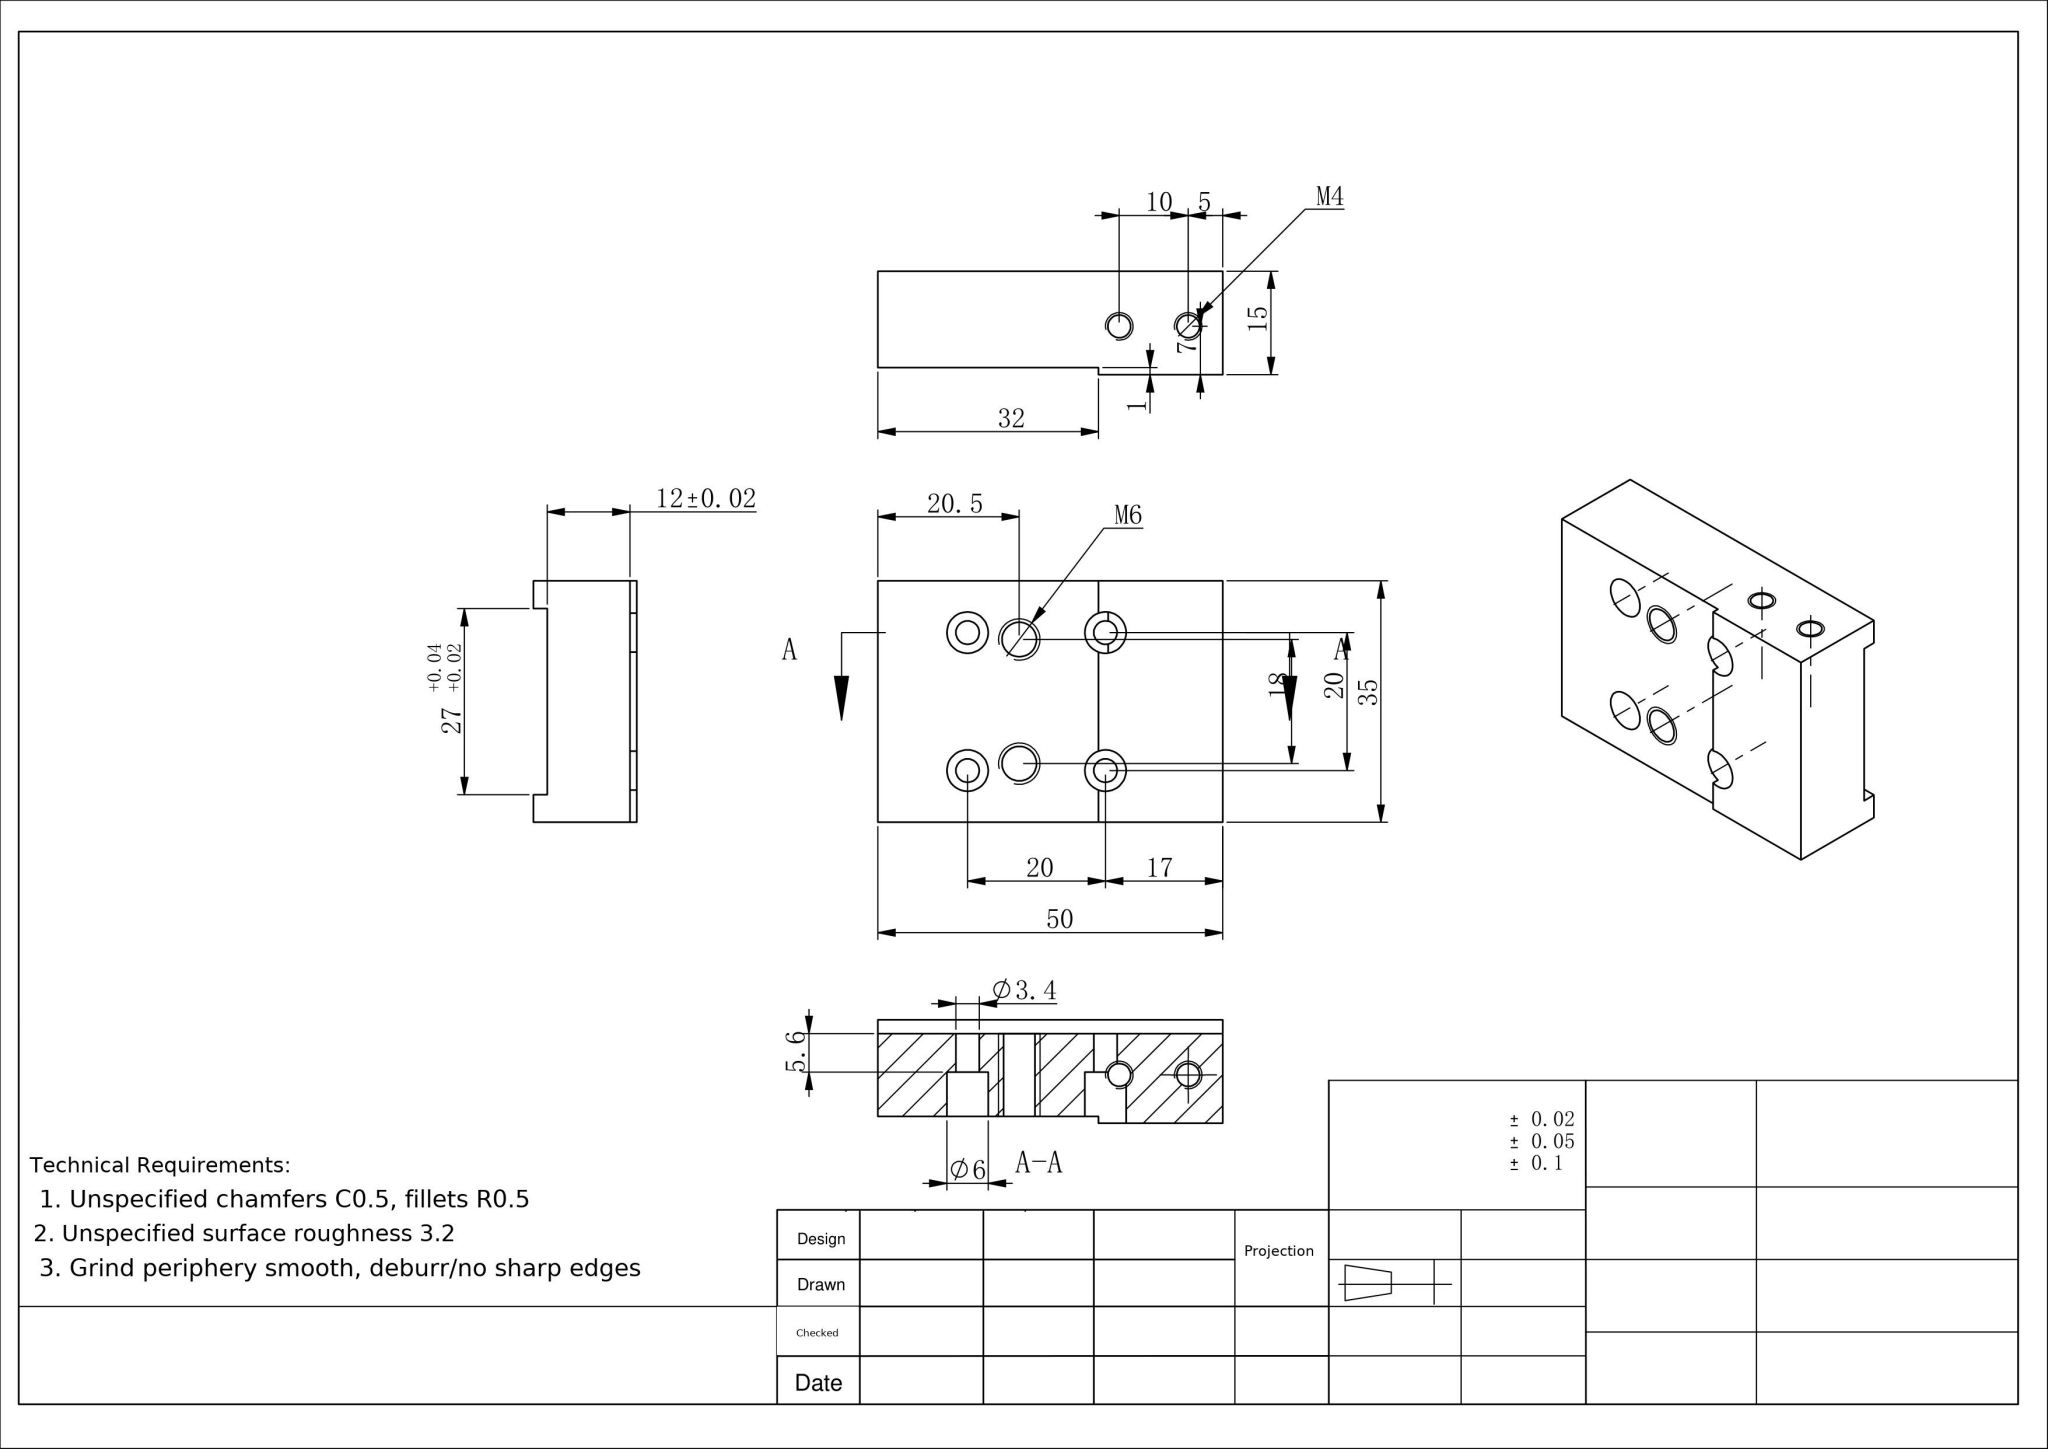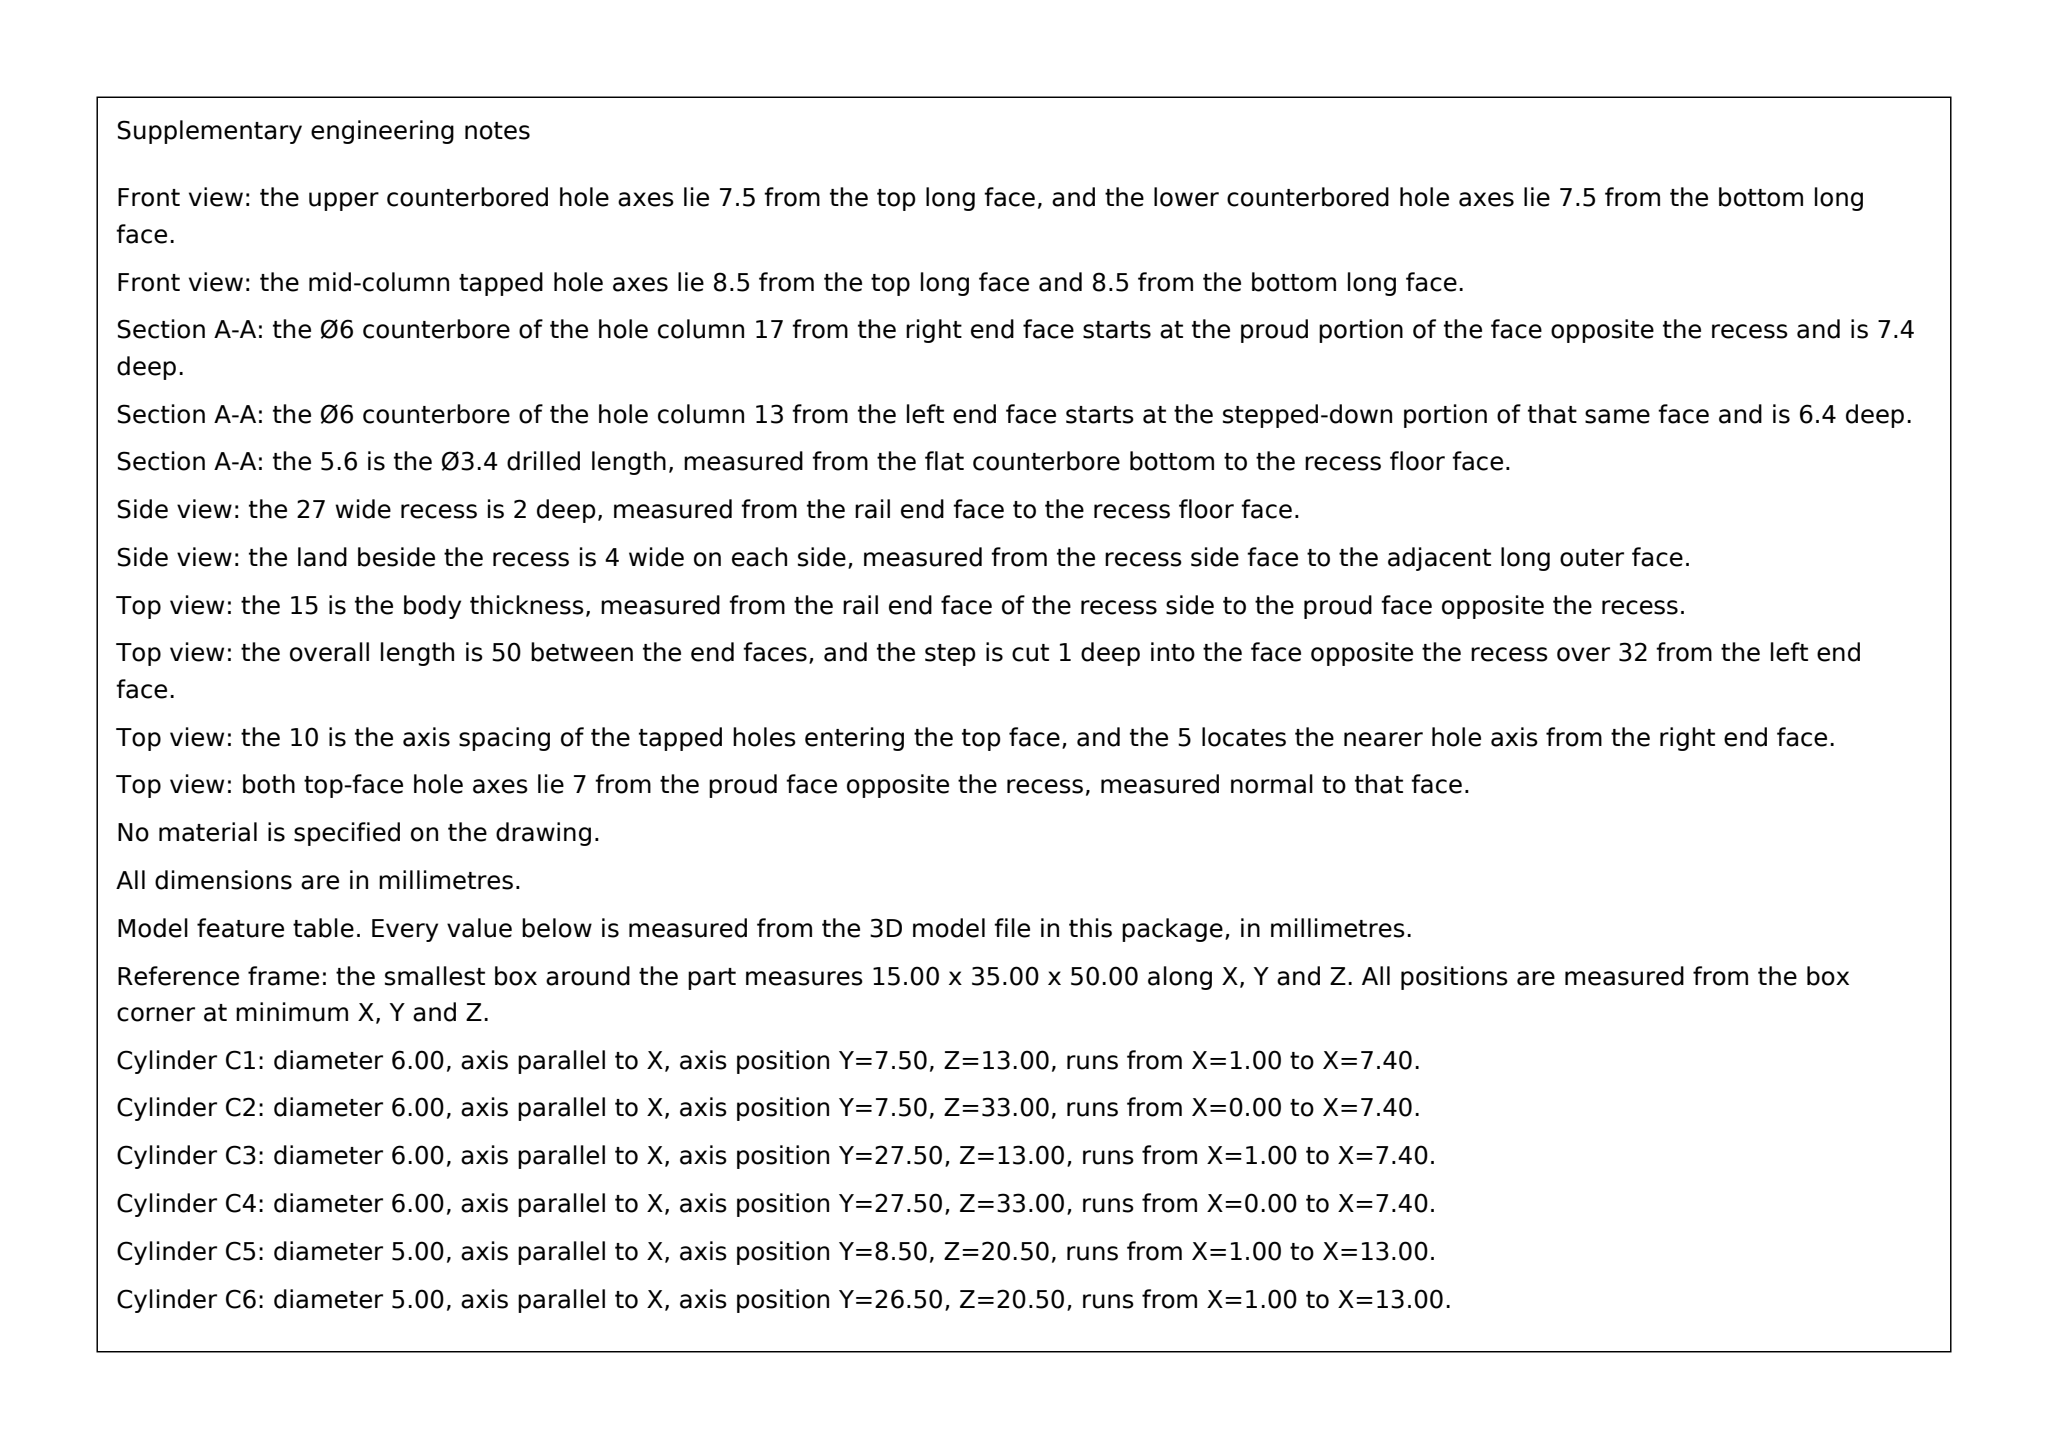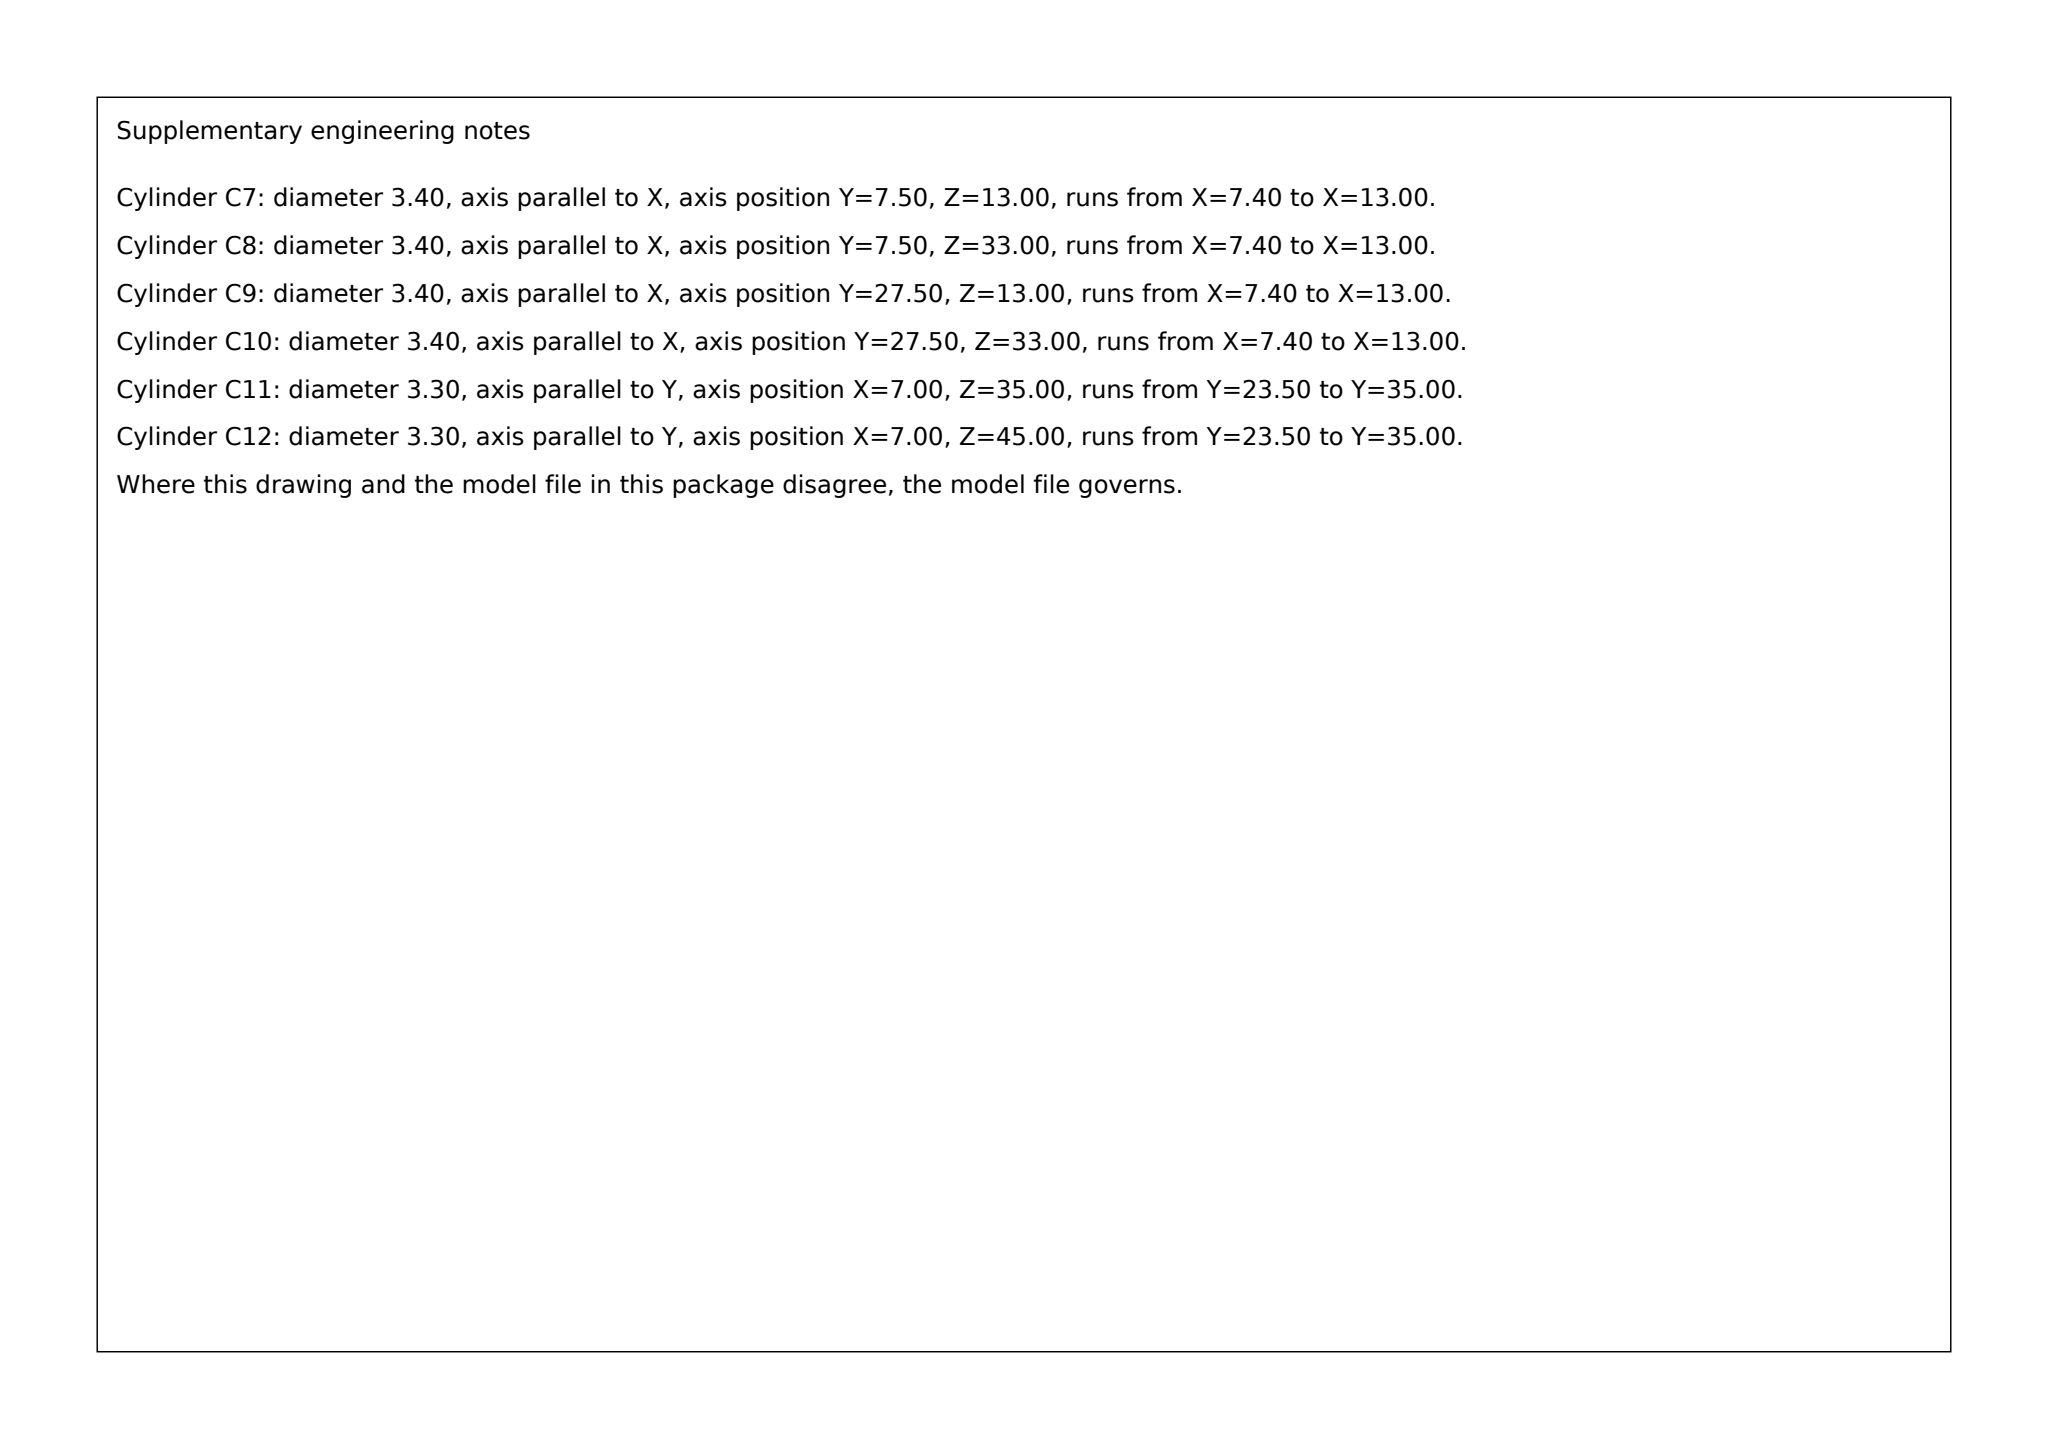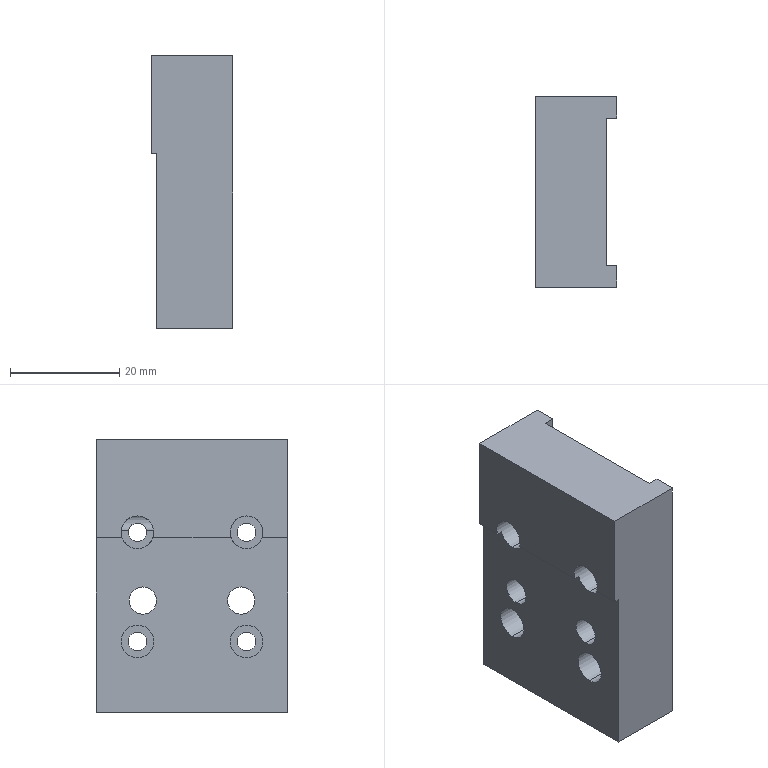Part | SolidWorks | mm | 1 solid | 46 faces | box 15 x 35 x 50 mm | volume 20813 mm3 | cylinder 24 | plane 18 | cone 4 | commonest cylinder face diameters 3.4 x8 6 x8 5 x4 3.3 x4
Drawing notes:
2X M6 DP 12, BLIND (Ø5 CORE) FROM FRONT FACE | from the solid: cylinders dia 5.0 axis x at y=8.5 & y=26.5, z=20.5, length 12.0 (blind, part 15 thick)
2X M4 DP 11.5, BLIND, FROM TONGUE TOP FACE | from the solid: cylinders dia 3.3 axis y at x=7.0, z=35 & z=45, length 11.5 with 118° drill point
A-A: 4X Ø6 C'BORE DP 6.4, Ø3.4 DP 5.6 BEYOND | from the solid: dia 6.0 bores length 6.4 (z=13) and 7.4 from x=0 at z=33 where face is at x=1.0, i.e. 6.4 deep from each c'bored face; dia 3.4 length 5.6
build123d program:
from build123d import *

# Parameters (mm, degrees)
SKETCH1_W                                            = 50
SKETCH1_H                                            = 35
BOSS_EXTRUDE1_DEPTH                                  = 15
SKETCH2_W                                            = 50
SKETCH2_H                                            = 27
CUT_EXTRUDE1_DEPTH                                   = 2
SKETCH17_W                                           = 32
SKETCH17_H                                           = 35
CUT_EXTRUDE3_DEPTH                                   = 1
HOLE_SIZE_ACCORDING_TO_THE_TYPE_OF_HEXAG_D           = 3.4
HOLE_SIZE_ACCORDING_TO_THE_TYPE_OF_HEXAG_CBORE_D     = 6
HOLE_SIZE_ACCORDING_TO_THE_TYPE_OF_HEXAG_CBORE_DEPTH = 7.4
M4_TAPPED_HOLE1_D                                    = 3.3
M4_TAPPED_HOLE1_DEPTH                                = 11.5
M4_TAPPED_HOLE1_TIP                                  = 0.9914
M6_TAPPED_HOLE1_D                                    = 5
M6_TAPPED_HOLE1_DEPTH                                = 17
M6_TAPPED_HOLE1_TIP                                  = 1.502


with BuildPart() as part:
    # Sketch1 → Boss-Extrude1 (new body)
    with BuildSketch(Plane(origin=(0, 0, 0), x_dir=(0, 0, -1), z_dir=(1, 0, 0))):
        Rectangle(SKETCH1_W, SKETCH1_H)
    extrude(amount=BOSS_EXTRUDE1_DEPTH)

    # Sketch2 → Cut-Extrude1 (cut)
    with BuildSketch(Plane(origin=(15, 0, 0), x_dir=(0, 0, -1), z_dir=(1, 0, 0))):
        Rectangle(SKETCH2_W, SKETCH2_H)
    extrude(amount=-CUT_EXTRUDE1_DEPTH, mode=Mode.SUBTRACT)

    # Sketch17 → Cut-Extrude3 (cut)
    with BuildSketch(Plane.ZY):
        with Locations((-9, 0)):
            Rectangle(SKETCH17_W, SKETCH17_H)
    extrude(amount=-CUT_EXTRUDE3_DEPTH, mode=Mode.SUBTRACT)

    # Hole Size according to the type of hexag (through all)
    with Locations(Plane.ZY):
        with Locations((8, 10), (8, -10), (-12, -10), (-12, 10)):
            CounterBoreHole(HOLE_SIZE_ACCORDING_TO_THE_TYPE_OF_HEXAG_D / 2, HOLE_SIZE_ACCORDING_TO_THE_TYPE_OF_HEXAG_CBORE_D / 2, HOLE_SIZE_ACCORDING_TO_THE_TYPE_OF_HEXAG_CBORE_DEPTH)

    # M4 Tapped Hole1
    with Locations(Plane(origin=(0, 17.5, 0), x_dir=(1, 0, 0), z_dir=(0, 1, 0))):
        with Locations((7, -20), (7, -10)):
            Hole(M4_TAPPED_HOLE1_D / 2, depth=M4_TAPPED_HOLE1_DEPTH)
            with Locations((0, 0, -(M4_TAPPED_HOLE1_DEPTH + M4_TAPPED_HOLE1_TIP / 2))):  # 118° drill point
                Cone(0, M4_TAPPED_HOLE1_D / 2, M4_TAPPED_HOLE1_TIP, mode=Mode.SUBTRACT)

    # M6 Tapped Hole1
    with Locations(Plane.ZY.offset(-1)):
        with Locations((-4.5, 9), (-4.5, -9)):
            Hole(M6_TAPPED_HOLE1_D / 2, depth=M6_TAPPED_HOLE1_DEPTH)
            with Locations((0, 0, -(M6_TAPPED_HOLE1_DEPTH + M6_TAPPED_HOLE1_TIP / 2))):  # 118° drill point
                Cone(0, M6_TAPPED_HOLE1_D / 2, M6_TAPPED_HOLE1_TIP, mode=Mode.SUBTRACT)


solid = part.part